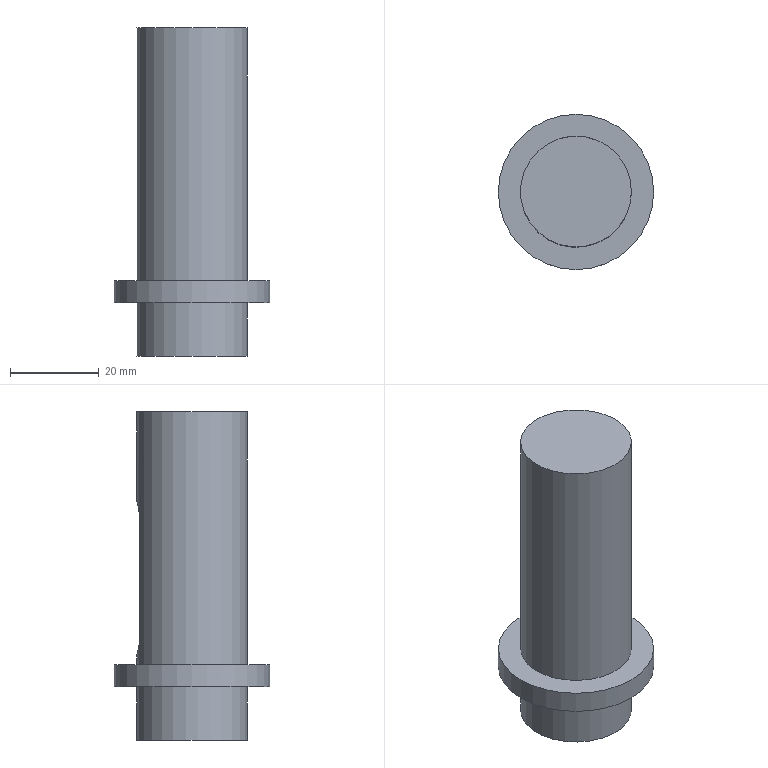Component | NX | MIDDLE_SHAFT | 1 solid | 12 faces | box 35 x 35 x 74 mm | volume 37671 mm3 | plane 7 | cylinder 5 | commonest cylinder face diameters 25 x2 8 x2 35 x1
STEP:
#1=CARTESIAN_POINT('',(0.,0.,0.));
#2=DIRECTION('',(0.,0.,1.));
#3=DIRECTION('',(1.,0.,0.));
#4=AXIS2_PLACEMENT_3D('',#1,#2,#3);
#5=CARTESIAN_POINT('',(-498.675,308.181,-737.));
#6=VERTEX_POINT('',#5);
#7=CARTESIAN_POINT('',(-511.175,308.181,-737.));
#8=DIRECTION('',(0.,0.,1.));
#9=DIRECTION('',(1.,0.,0.));
#10=AXIS2_PLACEMENT_3D('',#7,#8,#9);
#11=CIRCLE('',#10,12.5);
#12=CARTESIAN_POINT('',(-511.175,308.181,-737.));
#13=DIRECTION('',(0.,0.,-1.));
#14=DIRECTION('',(-1.,0.,0.));
#15=AXIS2_PLACEMENT_3D('',#12,#13,#14);
#16=PLANE('',#15);
#17=CARTESIAN_POINT('',(-12.5,0.));
#18=CARTESIAN_POINT('',(-12.5,21.651));
#19=CARTESIAN_POINT('',(6.25,10.825));
#20=CARTESIAN_POINT('',(25.,0.));
#21=CARTESIAN_POINT('',(6.25,-10.825));
#22=CARTESIAN_POINT('',(-12.5,-21.651));
#23=CARTESIAN_POINT('',(-12.5,0.));
#24=(BOUNDED_CURVE()B_SPLINE_CURVE(2,(#17,#18,#19,#20,#21,#22,#23),.UNSPECIFIED.,.T.,.F.)B_SPLINE_CURVE_WITH_KNOTS((1,2,2,2,2,1),(-2.094,0.,2.094,4.189,6.283,8.378),.UNSPECIFIED.)CURVE()GEOMETRIC_REPRESENTATION_ITEM()RATIONAL_B_SPLINE_CURVE((1.,0.5,1.,0.5,1.,0.5,1.))REPRESENTATION_ITEM(''));
#25=(GEOMETRIC_REPRESENTATION_CONTEXT(2)PARAMETRIC_REPRESENTATION_CONTEXT()REPRESENTATION_CONTEXT('',''));
#26=DEFINITIONAL_REPRESENTATION('',(#24),#25);
#27=PCURVE('',#16,#26);
#28=CARTESIAN_POINT('',(-511.175,308.181,-737.));
#29=DIRECTION('',(0.,0.,1.));
#30=DIRECTION('',(1.,0.,0.));
#31=AXIS2_PLACEMENT_3D('',#28,#29,#30);
#32=CYLINDRICAL_SURFACE('',#31,12.5);
#33=CARTESIAN_POINT('',(0.,0.));
#34=DIRECTION('',(1.,0.));
#35=VECTOR('',#34,1.);
#36=LINE('',#33,#35);
#37=(GEOMETRIC_REPRESENTATION_CONTEXT(2)PARAMETRIC_REPRESENTATION_CONTEXT()REPRESENTATION_CONTEXT('',''));
#38=DEFINITIONAL_REPRESENTATION('',(#36),#37);
#39=PCURVE('',#32,#38);
#40=SURFACE_CURVE('',#11,(#27,#39),.PCURVE_S1.);
#41=EDGE_CURVE('',#6,#6,#40,.T.);
#42=ORIENTED_EDGE('',*,*,#41,.F.);
#43=EDGE_LOOP('',(#42));
#44=FACE_BOUND('',#43,.T.);
#45=ADVANCED_FACE('',(#44),#16,.T.);
#46=CARTESIAN_POINT('',(-498.675,308.181,-725.));
#47=VERTEX_POINT('',#46);
#48=CARTESIAN_POINT('',(-511.175,308.181,-725.));
#49=DIRECTION('',(0.,0.,-1.));
#50=DIRECTION('',(1.,0.,0.));
#51=AXIS2_PLACEMENT_3D('',#48,#49,#50);
#52=CIRCLE('',#51,12.5);
#53=CARTESIAN_POINT('',(6.283,12.));
#54=DIRECTION('',(-1.,0.));
#55=VECTOR('',#54,1.);
#56=LINE('',#53,#55);
#57=(GEOMETRIC_REPRESENTATION_CONTEXT(2)PARAMETRIC_REPRESENTATION_CONTEXT()REPRESENTATION_CONTEXT('',''));
#58=DEFINITIONAL_REPRESENTATION('',(#56),#57);
#59=PCURVE('',#32,#58);
#60=CARTESIAN_POINT('',(-511.175,308.181,-725.));
#61=DIRECTION('',(0.,0.,1.));
#62=DIRECTION('',(1.,0.,0.));
#63=AXIS2_PLACEMENT_3D('',#60,#61,#62);
#64=PLANE('',#63);
#65=CARTESIAN_POINT('',(12.5,0.));
#66=CARTESIAN_POINT('',(12.5,-21.651));
#67=CARTESIAN_POINT('',(-6.25,-10.825));
#68=CARTESIAN_POINT('',(-25.,-0.));
#69=CARTESIAN_POINT('',(-6.25,10.825));
#70=CARTESIAN_POINT('',(12.5,21.651));
#71=CARTESIAN_POINT('',(12.5,0.));
#72=(BOUNDED_CURVE()B_SPLINE_CURVE(2,(#65,#66,#67,#68,#69,#70,#71),.UNSPECIFIED.,.T.,.F.)B_SPLINE_CURVE_WITH_KNOTS((1,2,2,2,2,1),(-2.094,0.,2.094,4.189,6.283,8.378),.UNSPECIFIED.)CURVE()GEOMETRIC_REPRESENTATION_ITEM()RATIONAL_B_SPLINE_CURVE((1.,0.5,1.,0.5,1.,0.5,1.))REPRESENTATION_ITEM(''));
#73=(GEOMETRIC_REPRESENTATION_CONTEXT(2)PARAMETRIC_REPRESENTATION_CONTEXT()REPRESENTATION_CONTEXT('',''));
#74=DEFINITIONAL_REPRESENTATION('',(#72),#73);
#75=PCURVE('',#64,#74);
#76=SURFACE_CURVE('',#52,(#59,#75),.PCURVE_S1.);
#77=EDGE_CURVE('',#47,#47,#76,.T.);
#78=ORIENTED_EDGE('',*,*,#77,.T.);
#79=CARTESIAN_POINT('',(-498.675,308.181,-737.));
#80=CARTESIAN_POINT('',(-498.675,308.181,-725.));
#81=B_SPLINE_CURVE_WITH_KNOTS('',1,(#79,#80),.UNSPECIFIED.,.F.,.F.,(2,2),(0.,12.),.PIECEWISE_BEZIER_KNOTS.);
#82=CARTESIAN_POINT('',(0.,0.));
#83=DIRECTION('',(0.,1.));
#84=VECTOR('',#83,1.);
#85=LINE('',#82,#84);
#86=(GEOMETRIC_REPRESENTATION_CONTEXT(2)PARAMETRIC_REPRESENTATION_CONTEXT()REPRESENTATION_CONTEXT('',''));
#87=DEFINITIONAL_REPRESENTATION('',(#85),#86);
#88=PCURVE('',#32,#87);
#89=CARTESIAN_POINT('',(6.283,0.));
#90=DIRECTION('',(0.,1.));
#91=VECTOR('',#90,1.);
#92=LINE('',#89,#91);
#93=(GEOMETRIC_REPRESENTATION_CONTEXT(2)PARAMETRIC_REPRESENTATION_CONTEXT()REPRESENTATION_CONTEXT('',''));
#94=DEFINITIONAL_REPRESENTATION('',(#92),#93);
#95=PCURVE('',#32,#94);
#96=SEAM_CURVE('',#81,(#88,#95),.PCURVE_S1.);
#97=EDGE_CURVE('',#6,#47,#96,.T.);
#98=ORIENTED_EDGE('',*,*,#97,.F.);
#99=ORIENTED_EDGE('',*,*,#41,.T.);
#100=ORIENTED_EDGE('',*,*,#97,.T.);
#101=EDGE_LOOP('',(#78,#98,#99,#100));
#102=FACE_BOUND('',#101,.T.);
#103=ADVANCED_FACE('',(#102),#32,.T.);
#104=CARTESIAN_POINT('',(-493.675,308.181,-720.));
#105=VERTEX_POINT('',#104);
#106=CARTESIAN_POINT('',(-511.175,308.181,-720.));
#107=DIRECTION('',(0.,0.,1.));
#108=DIRECTION('',(1.,0.,0.));
#109=AXIS2_PLACEMENT_3D('',#106,#107,#108);
#110=CIRCLE('',#109,17.5);
#111=CARTESIAN_POINT('',(-511.175,308.181,-720.));
#112=DIRECTION('',(0.,0.,-1.));
#113=DIRECTION('',(-1.,0.,0.));
#114=AXIS2_PLACEMENT_3D('',#111,#112,#113);
#115=CYLINDRICAL_SURFACE('',#114,17.5);
#116=CARTESIAN_POINT('',(9.425,0.));
#117=DIRECTION('',(-1.,0.));
#118=VECTOR('',#117,1.);
#119=LINE('',#116,#118);
#120=(GEOMETRIC_REPRESENTATION_CONTEXT(2)PARAMETRIC_REPRESENTATION_CONTEXT()REPRESENTATION_CONTEXT('',''));
#121=DEFINITIONAL_REPRESENTATION('',(#119),#120);
#122=PCURVE('',#115,#121);
#123=CARTESIAN_POINT('',(-511.175,308.181,-720.));
#124=DIRECTION('',(0.,0.,1.));
#125=DIRECTION('',(1.,0.,0.));
#126=AXIS2_PLACEMENT_3D('',#123,#124,#125);
#127=PLANE('',#126);
#128=CARTESIAN_POINT('',(0.,0.));
#129=DIRECTION('',(1.,0.));
#130=AXIS2_PLACEMENT_2D('',#128,#129);
#131=CIRCLE('',#130,17.5);
#132=(GEOMETRIC_REPRESENTATION_CONTEXT(2)PARAMETRIC_REPRESENTATION_CONTEXT()REPRESENTATION_CONTEXT('',''));
#133=DEFINITIONAL_REPRESENTATION('',(#131),#132);
#134=PCURVE('',#127,#133);
#135=SURFACE_CURVE('',#110,(#122,#134),.PCURVE_S1.);
#136=EDGE_CURVE('',#105,#105,#135,.T.);
#137=ORIENTED_EDGE('',*,*,#136,.F.);
#138=CARTESIAN_POINT('',(-493.675,308.181,-725.));
#139=VERTEX_POINT('',#138);
#140=CARTESIAN_POINT('',(-493.675,308.181,-720.));
#141=CARTESIAN_POINT('',(-493.675,308.181,-725.));
#142=B_SPLINE_CURVE_WITH_KNOTS('',1,(#140,#141),.UNSPECIFIED.,.F.,.F.,(2,2),(0.,5.),.PIECEWISE_BEZIER_KNOTS.);
#143=CARTESIAN_POINT('',(9.425,0.));
#144=DIRECTION('',(0.,1.));
#145=VECTOR('',#144,1.);
#146=LINE('',#143,#145);
#147=(GEOMETRIC_REPRESENTATION_CONTEXT(2)PARAMETRIC_REPRESENTATION_CONTEXT()REPRESENTATION_CONTEXT('',''));
#148=DEFINITIONAL_REPRESENTATION('',(#146),#147);
#149=PCURVE('',#115,#148);
#150=CARTESIAN_POINT('',(3.142,0.));
#151=DIRECTION('',(0.,1.));
#152=VECTOR('',#151,1.);
#153=LINE('',#150,#152);
#154=(GEOMETRIC_REPRESENTATION_CONTEXT(2)PARAMETRIC_REPRESENTATION_CONTEXT()REPRESENTATION_CONTEXT('',''));
#155=DEFINITIONAL_REPRESENTATION('',(#153),#154);
#156=PCURVE('',#115,#155);
#157=SEAM_CURVE('',#142,(#149,#156),.PCURVE_S1.);
#158=EDGE_CURVE('',#105,#139,#157,.T.);
#159=ORIENTED_EDGE('',*,*,#158,.T.);
#160=CARTESIAN_POINT('',(-511.175,308.181,-725.));
#161=DIRECTION('',(0.,0.,1.));
#162=DIRECTION('',(1.,0.,0.));
#163=AXIS2_PLACEMENT_3D('',#160,#161,#162);
#164=CIRCLE('',#163,17.5);
#165=CARTESIAN_POINT('',(9.425,5.));
#166=DIRECTION('',(-1.,0.));
#167=VECTOR('',#166,1.);
#168=LINE('',#165,#167);
#169=(GEOMETRIC_REPRESENTATION_CONTEXT(2)PARAMETRIC_REPRESENTATION_CONTEXT()REPRESENTATION_CONTEXT('',''));
#170=DEFINITIONAL_REPRESENTATION('',(#168),#169);
#171=PCURVE('',#115,#170);
#172=CARTESIAN_POINT('',(0.,0.));
#173=DIRECTION('',(1.,0.));
#174=AXIS2_PLACEMENT_2D('',#172,#173);
#175=CIRCLE('',#174,17.5);
#176=(GEOMETRIC_REPRESENTATION_CONTEXT(2)PARAMETRIC_REPRESENTATION_CONTEXT()REPRESENTATION_CONTEXT('',''));
#177=DEFINITIONAL_REPRESENTATION('',(#175),#176);
#178=PCURVE('',#64,#177);
#179=SURFACE_CURVE('',#164,(#171,#178),.PCURVE_S1.);
#180=EDGE_CURVE('',#139,#139,#179,.T.);
#181=ORIENTED_EDGE('',*,*,#180,.T.);
#182=ORIENTED_EDGE('',*,*,#158,.F.);
#183=EDGE_LOOP('',(#137,#159,#181,#182));
#184=FACE_BOUND('',#183,.T.);
#185=ADVANCED_FACE('',(#184),#115,.T.);
#186=CARTESIAN_POINT('',(-498.675,308.181,-720.));
#187=VERTEX_POINT('',#186);
#188=CARTESIAN_POINT('',(-511.175,308.181,-720.));
#189=DIRECTION('',(0.,0.,1.));
#190=DIRECTION('',(1.,0.,0.));
#191=AXIS2_PLACEMENT_3D('',#188,#189,#190);
#192=CIRCLE('',#191,12.5);
#193=CARTESIAN_POINT('',(0.,0.));
#194=DIRECTION('',(1.,0.));
#195=AXIS2_PLACEMENT_2D('',#193,#194);
#196=CIRCLE('',#195,12.5);
#197=(GEOMETRIC_REPRESENTATION_CONTEXT(2)PARAMETRIC_REPRESENTATION_CONTEXT()REPRESENTATION_CONTEXT('',''));
#198=DEFINITIONAL_REPRESENTATION('',(#196),#197);
#199=PCURVE('',#127,#198);
#200=CARTESIAN_POINT('',(-511.175,308.181,-720.));
#201=DIRECTION('',(0.,0.,1.));
#202=DIRECTION('',(1.,0.,0.));
#203=AXIS2_PLACEMENT_3D('',#200,#201,#202);
#204=CYLINDRICAL_SURFACE('',#203,12.5);
#205=CARTESIAN_POINT('',(0.,0.));
#206=DIRECTION('',(1.,0.));
#207=VECTOR('',#206,1.);
#208=LINE('',#205,#207);
#209=(GEOMETRIC_REPRESENTATION_CONTEXT(2)PARAMETRIC_REPRESENTATION_CONTEXT()REPRESENTATION_CONTEXT('',''));
#210=DEFINITIONAL_REPRESENTATION('',(#208),#209);
#211=PCURVE('',#204,#210);
#212=SURFACE_CURVE('',#192,(#199,#211),.PCURVE_S1.);
#213=EDGE_CURVE('',#187,#187,#212,.T.);
#214=ORIENTED_EDGE('',*,*,#213,.F.);
#215=EDGE_LOOP('',(#214));
#216=FACE_BOUND('',#215,.T.);
#217=ORIENTED_EDGE('',*,*,#136,.T.);
#218=EDGE_LOOP('',(#217));
#219=FACE_BOUND('',#218,.T.);
#220=ADVANCED_FACE('',(#216,#219),#127,.T.);
#221=ORIENTED_EDGE('',*,*,#77,.F.);
#222=EDGE_LOOP('',(#221));
#223=FACE_BOUND('',#222,.T.);
#224=ORIENTED_EDGE('',*,*,#180,.F.);
#225=EDGE_LOOP('',(#224));
#226=FACE_BOUND('',#225,.T.);
#227=ADVANCED_FACE('',(#223,#226),#64,.F.);
#228=CARTESIAN_POINT('',(-498.675,308.181,-663.));
#229=VERTEX_POINT('',#228);
#230=CARTESIAN_POINT('',(-511.175,308.181,-663.));
#231=DIRECTION('',(0.,0.,-1.));
#232=DIRECTION('',(1.,0.,0.));
#233=AXIS2_PLACEMENT_3D('',#230,#231,#232);
#234=CIRCLE('',#233,12.5);
#235=CARTESIAN_POINT('',(-511.175,308.181,-663.));
#236=DIRECTION('',(0.,0.,1.));
#237=DIRECTION('',(1.,0.,0.));
#238=AXIS2_PLACEMENT_3D('',#235,#236,#237);
#239=PLANE('',#238);
#240=CARTESIAN_POINT('',(12.5,0.));
#241=CARTESIAN_POINT('',(12.5,-21.651));
#242=CARTESIAN_POINT('',(-6.25,-10.825));
#243=CARTESIAN_POINT('',(-25.,-0.));
#244=CARTESIAN_POINT('',(-6.25,10.825));
#245=CARTESIAN_POINT('',(12.5,21.651));
#246=CARTESIAN_POINT('',(12.5,0.));
#247=(BOUNDED_CURVE()B_SPLINE_CURVE(2,(#240,#241,#242,#243,#244,#245,#246),.UNSPECIFIED.,.T.,.F.)B_SPLINE_CURVE_WITH_KNOTS((1,2,2,2,2,1),(-2.094,0.,2.094,4.189,6.283,8.378),.UNSPECIFIED.)CURVE()GEOMETRIC_REPRESENTATION_ITEM()RATIONAL_B_SPLINE_CURVE((1.,0.5,1.,0.5,1.,0.5,1.))REPRESENTATION_ITEM(''));
#248=(GEOMETRIC_REPRESENTATION_CONTEXT(2)PARAMETRIC_REPRESENTATION_CONTEXT()REPRESENTATION_CONTEXT('',''));
#249=DEFINITIONAL_REPRESENTATION('',(#247),#248);
#250=PCURVE('',#239,#249);
#251=CARTESIAN_POINT('',(6.283,57.));
#252=DIRECTION('',(-1.,0.));
#253=VECTOR('',#252,1.);
#254=LINE('',#251,#253);
#255=(GEOMETRIC_REPRESENTATION_CONTEXT(2)PARAMETRIC_REPRESENTATION_CONTEXT()REPRESENTATION_CONTEXT('',''));
#256=DEFINITIONAL_REPRESENTATION('',(#254),#255);
#257=PCURVE('',#204,#256);
#258=SURFACE_CURVE('',#234,(#250,#257),.PCURVE_S1.);
#259=EDGE_CURVE('',#229,#229,#258,.T.);
#260=ORIENTED_EDGE('',*,*,#259,.F.);
#261=EDGE_LOOP('',(#260));
#262=FACE_BOUND('',#261,.T.);
#263=ADVANCED_FACE('',(#262),#239,.T.);
#264=ORIENTED_EDGE('',*,*,#259,.T.);
#265=CARTESIAN_POINT('',(-498.675,308.181,-720.));
#266=CARTESIAN_POINT('',(-498.675,308.181,-663.));
#267=B_SPLINE_CURVE_WITH_KNOTS('',1,(#265,#266),.UNSPECIFIED.,.F.,.F.,(2,2),(0.,57.),.PIECEWISE_BEZIER_KNOTS.);
#268=CARTESIAN_POINT('',(0.,0.));
#269=DIRECTION('',(0.,1.));
#270=VECTOR('',#269,1.);
#271=LINE('',#268,#270);
#272=(GEOMETRIC_REPRESENTATION_CONTEXT(2)PARAMETRIC_REPRESENTATION_CONTEXT()REPRESENTATION_CONTEXT('',''));
#273=DEFINITIONAL_REPRESENTATION('',(#271),#272);
#274=PCURVE('',#204,#273);
#275=CARTESIAN_POINT('',(6.283,0.));
#276=DIRECTION('',(0.,1.));
#277=VECTOR('',#276,1.);
#278=LINE('',#275,#277);
#279=(GEOMETRIC_REPRESENTATION_CONTEXT(2)PARAMETRIC_REPRESENTATION_CONTEXT()REPRESENTATION_CONTEXT('',''));
#280=DEFINITIONAL_REPRESENTATION('',(#278),#279);
#281=PCURVE('',#204,#280);
#282=SEAM_CURVE('',#267,(#274,#281),.PCURVE_S1.);
#283=EDGE_CURVE('',#187,#229,#282,.T.);
#284=ORIENTED_EDGE('',*,*,#283,.F.);
#285=ORIENTED_EDGE('',*,*,#213,.T.);
#286=ORIENTED_EDGE('',*,*,#283,.T.);
#287=EDGE_LOOP('',(#264,#284,#285,#286));
#288=FACE_BOUND('',#287,.T.);
#289=CARTESIAN_POINT('',(-507.175,320.024,-687.));
#290=VERTEX_POINT('',#289);
#291=CARTESIAN_POINT('',(-507.175,320.024,-714.));
#292=VERTEX_POINT('',#291);
#293=CARTESIAN_POINT('',(-507.175,320.024,-720.));
#294=DIRECTION('',(0.,0.,-1.));
#295=VECTOR('',#294,1.);
#296=LINE('',#293,#295);
#297=CARTESIAN_POINT('',(1.245,0.));
#298=DIRECTION('',(0.,-1.));
#299=VECTOR('',#298,1.);
#300=LINE('',#297,#299);
#301=(GEOMETRIC_REPRESENTATION_CONTEXT(2)PARAMETRIC_REPRESENTATION_CONTEXT()REPRESENTATION_CONTEXT('',''));
#302=DEFINITIONAL_REPRESENTATION('',(#300),#301);
#303=PCURVE('',#204,#302);
#304=CARTESIAN_POINT('',(-507.175,308.181,-737.));
#305=DIRECTION('',(1.,0.,0.));
#306=DIRECTION('',(0.,0.,-1.));
#307=AXIS2_PLACEMENT_3D('',#304,#305,#306);
#308=PLANE('',#307);
#309=CARTESIAN_POINT('',(-17.,11.843));
#310=DIRECTION('',(1.,0.));
#311=VECTOR('',#310,1.);
#312=LINE('',#309,#311);
#313=(GEOMETRIC_REPRESENTATION_CONTEXT(2)PARAMETRIC_REPRESENTATION_CONTEXT()REPRESENTATION_CONTEXT('',''));
#314=DEFINITIONAL_REPRESENTATION('',(#312),#313);
#315=PCURVE('',#308,#314);
#316=SURFACE_CURVE('',#296,(#303,#315),.PCURVE_S1.);
#317=EDGE_CURVE('',#290,#292,#316,.T.);
#318=ORIENTED_EDGE('',*,*,#317,.F.);
#319=CARTESIAN_POINT('',(-515.175,320.024,-687.));
#320=VERTEX_POINT('',#319);
#321=CARTESIAN_POINT('',(-507.175,320.024,-687.));
#322=CARTESIAN_POINT('',(-507.175,320.024,-686.565));
#323=CARTESIAN_POINT('',(-507.248,320.049,-686.125));
#324=CARTESIAN_POINT('',(-507.387,320.094,-685.715));
#325=CARTESIAN_POINT('',(-507.526,320.138,-685.306));
#326=CARTESIAN_POINT('',(-507.734,320.201,-684.917));
#327=CARTESIAN_POINT('',(-507.994,320.27,-684.576));
#328=CARTESIAN_POINT('',(-508.262,320.34,-684.223));
#329=CARTESIAN_POINT('',(-508.593,320.418,-683.913));
#330=CARTESIAN_POINT('',(-508.963,320.484,-683.668));
#331=CARTESIAN_POINT('',(-509.341,320.552,-683.417));
#332=CARTESIAN_POINT('',(-509.77,320.61,-683.227));
#333=CARTESIAN_POINT('',(-510.215,320.644,-683.117));
#334=CARTESIAN_POINT('',(-510.527,320.668,-683.04));
#335=CARTESIAN_POINT('',(-510.852,320.681,-683.));
#336=CARTESIAN_POINT('',(-511.175,320.681,-683.));
#337=CARTESIAN_POINT('',(-511.611,320.681,-683.));
#338=CARTESIAN_POINT('',(-512.052,320.657,-683.073));
#339=CARTESIAN_POINT('',(-512.462,320.615,-683.213));
#340=CARTESIAN_POINT('',(-512.872,320.573,-683.352));
#341=CARTESIAN_POINT('',(-513.262,320.511,-683.561));
#342=CARTESIAN_POINT('',(-513.604,320.443,-683.821));
#343=CARTESIAN_POINT('',(-513.955,320.374,-684.09));
#344=CARTESIAN_POINT('',(-514.265,320.296,-684.421));
#345=CARTESIAN_POINT('',(-514.509,320.229,-684.79));
#346=CARTESIAN_POINT('',(-514.76,320.159,-685.168));
#347=CARTESIAN_POINT('',(-514.949,320.099,-685.597));
#348=CARTESIAN_POINT('',(-515.059,320.063,-686.041));
#349=CARTESIAN_POINT('',(-515.136,320.038,-686.353));
#350=CARTESIAN_POINT('',(-515.175,320.024,-686.678));
#351=CARTESIAN_POINT('',(-515.175,320.024,-687.));
#352=B_SPLINE_CURVE_WITH_KNOTS('',3,(#321,#322,#323,#324,#325,#326,#327,#328,#329,#330,#331,#332,#333,#334,#335,#336,#337,#338,#339,#340,#341,#342,#343,#344,#345,#346,#347,#348,#349,#350,#351),.UNSPECIFIED.,.F.,.F.,(4,3,3,3,3,3,3,3,3,3,4),(0.,0.1037,0.2071,0.314,0.4235,0.5,0.6038,0.7074,0.8141,0.9237,1.),.UNSPECIFIED.);
#353=CARTESIAN_POINT('',(1.245,33.));
#354=CARTESIAN_POINT('',(1.245,33.095));
#355=CARTESIAN_POINT('',(1.246,33.286));
#356=CARTESIAN_POINT('',(1.248,33.573));
#357=CARTESIAN_POINT('',(1.253,33.856));
#358=CARTESIAN_POINT('',(1.259,34.134));
#359=CARTESIAN_POINT('',(1.266,34.404));
#360=CARTESIAN_POINT('',(1.275,34.667));
#361=CARTESIAN_POINT('',(1.286,34.923));
#362=CARTESIAN_POINT('',(1.298,35.168));
#363=CARTESIAN_POINT('',(1.312,35.401));
#364=CARTESIAN_POINT('',(1.326,35.621));
#365=CARTESIAN_POINT('',(1.342,35.829));
#366=CARTESIAN_POINT('',(1.359,36.023));
#367=CARTESIAN_POINT('',(1.377,36.202));
#368=CARTESIAN_POINT('',(1.396,36.364));
#369=CARTESIAN_POINT('',(1.416,36.509));
#370=CARTESIAN_POINT('',(1.437,36.637));
#371=CARTESIAN_POINT('',(1.458,36.747));
#372=CARTESIAN_POINT('',(1.48,36.839));
#373=CARTESIAN_POINT('',(1.502,36.91));
#374=CARTESIAN_POINT('',(1.525,36.962));
#375=CARTESIAN_POINT('',(1.548,36.993));
#376=CARTESIAN_POINT('',(1.571,37.004));
#377=CARTESIAN_POINT('',(1.594,36.993));
#378=CARTESIAN_POINT('',(1.617,36.962));
#379=CARTESIAN_POINT('',(1.639,36.91));
#380=CARTESIAN_POINT('',(1.662,36.839));
#381=CARTESIAN_POINT('',(1.683,36.749));
#382=CARTESIAN_POINT('',(1.705,36.639));
#383=CARTESIAN_POINT('',(1.725,36.511));
#384=CARTESIAN_POINT('',(1.745,36.365));
#385=CARTESIAN_POINT('',(1.764,36.203));
#386=CARTESIAN_POINT('',(1.782,36.025));
#387=CARTESIAN_POINT('',(1.799,35.831));
#388=CARTESIAN_POINT('',(1.815,35.623));
#389=CARTESIAN_POINT('',(1.83,35.402));
#390=CARTESIAN_POINT('',(1.843,35.17));
#391=CARTESIAN_POINT('',(1.855,34.926));
#392=CARTESIAN_POINT('',(1.866,34.671));
#393=CARTESIAN_POINT('',(1.875,34.407));
#394=CARTESIAN_POINT('',(1.883,34.136));
#395=CARTESIAN_POINT('',(1.889,33.86));
#396=CARTESIAN_POINT('',(1.893,33.576));
#397=CARTESIAN_POINT('',(1.896,33.288));
#398=CARTESIAN_POINT('',(1.897,33.096));
#399=CARTESIAN_POINT('',(1.897,33.));
#400=B_SPLINE_CURVE_WITH_KNOTS('',3,(#353,#354,#355,#356,#357,#358,#359,#360,#361,#362,#363,#364,#365,#366,#367,#368,#369,#370,#371,#372,#373,#374,#375,#376,#377,#378,#379,#380,#381,#382,#383,#384,#385,#386,#387,#388,#389,#390,#391,#392,#393,#394,#395,#396,#397,#398,#399),.UNSPECIFIED.,.F.,.F.,(4,1,1,1,1,1,1,1,1,1,1,1,1,1,1,1,1,1,1,1,1,1,1,1,1,1,1,1,1,1,1,1,1,1,1,1,1,1,1,1,1,1,1,1,4),(0.,0.02273,0.04545,0.06818,0.09091,0.1136,0.1364,0.1591,0.1818,0.2045,0.2273,0.25,0.2727,0.2955,0.3182,0.3409,0.3636,0.3864,0.4091,0.4318,0.4545,0.4773,0.5,0.5227,0.5455,0.5682,0.5909,0.6136,0.6364,0.6591,0.6818,0.7045,0.7273,0.75,0.7727,0.7955,0.8182,0.8409,0.8636,0.8864,0.9091,0.9318,0.9545,0.9773,1.),.QUASI_UNIFORM_KNOTS.);
#401=(GEOMETRIC_REPRESENTATION_CONTEXT(2)PARAMETRIC_REPRESENTATION_CONTEXT()REPRESENTATION_CONTEXT('',''));
#402=DEFINITIONAL_REPRESENTATION('',(#400),#401);
#403=PCURVE('',#204,#402);
#404=CARTESIAN_POINT('',(-511.175,308.181,-687.));
#405=DIRECTION('',(0.,1.,0.));
#406=DIRECTION('',(0.,0.,1.));
#407=AXIS2_PLACEMENT_3D('',#404,#405,#406);
#408=CYLINDRICAL_SURFACE('',#407,4.);
#409=CARTESIAN_POINT('',(1.571,11.843));
#410=CARTESIAN_POINT('',(1.547,11.843));
#411=CARTESIAN_POINT('',(1.499,11.845));
#412=CARTESIAN_POINT('',(1.427,11.856));
#413=CARTESIAN_POINT('',(1.355,11.873));
#414=CARTESIAN_POINT('',(1.284,11.896));
#415=CARTESIAN_POINT('',(1.213,11.925));
#416=CARTESIAN_POINT('',(1.141,11.959));
#417=CARTESIAN_POINT('',(1.07,11.997));
#418=CARTESIAN_POINT('',(0.9985,12.039));
#419=CARTESIAN_POINT('',(0.9276,12.083));
#420=CARTESIAN_POINT('',(0.857,12.129));
#421=CARTESIAN_POINT('',(0.7859,12.175));
#422=CARTESIAN_POINT('',(0.7149,12.222));
#423=CARTESIAN_POINT('',(0.6438,12.268));
#424=CARTESIAN_POINT('',(0.5731,12.311));
#425=CARTESIAN_POINT('',(0.5022,12.351));
#426=CARTESIAN_POINT('',(0.4308,12.388));
#427=CARTESIAN_POINT('',(0.3593,12.421));
#428=CARTESIAN_POINT('',(0.2878,12.449));
#429=CARTESIAN_POINT('',(0.2165,12.471));
#430=CARTESIAN_POINT('',(0.1443,12.488));
#431=CARTESIAN_POINT('',(0.07209,12.498));
#432=CARTESIAN_POINT('',(-0.0001412,12.501));
#433=CARTESIAN_POINT('',(-0.07158,12.498));
#434=CARTESIAN_POINT('',(-0.1436,12.488));
#435=CARTESIAN_POINT('',(-0.2155,12.472));
#436=CARTESIAN_POINT('',(-0.2872,12.449));
#437=CARTESIAN_POINT('',(-0.3583,12.422));
#438=CARTESIAN_POINT('',(-0.4297,12.389));
#439=CARTESIAN_POINT('',(-0.5012,12.352));
#440=CARTESIAN_POINT('',(-0.5725,12.311));
#441=CARTESIAN_POINT('',(-0.6434,12.268));
#442=CARTESIAN_POINT('',(-0.7141,12.223));
#443=CARTESIAN_POINT('',(-0.7851,12.176));
#444=CARTESIAN_POINT('',(-0.8562,12.129));
#445=CARTESIAN_POINT('',(-0.9272,12.083));
#446=CARTESIAN_POINT('',(-0.9979,12.039));
#447=CARTESIAN_POINT('',(-1.069,11.998));
#448=CARTESIAN_POINT('',(-1.14,11.959));
#449=CARTESIAN_POINT('',(-1.212,11.925));
#450=CARTESIAN_POINT('',(-1.283,11.896));
#451=CARTESIAN_POINT('',(-1.354,11.873));
#452=CARTESIAN_POINT('',(-1.427,11.856));
#453=CARTESIAN_POINT('',(-1.499,11.845));
#454=CARTESIAN_POINT('',(-1.547,11.843));
#455=CARTESIAN_POINT('',(-1.571,11.843));
#456=B_SPLINE_CURVE_WITH_KNOTS('',3,(#409,#410,#411,#412,#413,#414,#415,#416,#417,#418,#419,#420,#421,#422,#423,#424,#425,#426,#427,#428,#429,#430,#431,#432,#433,#434,#435,#436,#437,#438,#439,#440,#441,#442,#443,#444,#445,#446,#447,#448,#449,#450,#451,#452,#453,#454,#455),.UNSPECIFIED.,.F.,.F.,(4,1,1,1,1,1,1,1,1,1,1,1,1,1,1,1,1,1,1,1,1,1,1,1,1,1,1,1,1,1,1,1,1,1,1,1,1,1,1,1,1,1,1,1,4),(0.,0.02273,0.04545,0.06818,0.09091,0.1136,0.1364,0.1591,0.1818,0.2045,0.2273,0.25,0.2727,0.2955,0.3182,0.3409,0.3636,0.3864,0.4091,0.4318,0.4545,0.4773,0.5,0.5227,0.5455,0.5682,0.5909,0.6136,0.6364,0.6591,0.6818,0.7045,0.7273,0.75,0.7727,0.7955,0.8182,0.8409,0.8636,0.8864,0.9091,0.9318,0.9545,0.9773,1.),.QUASI_UNIFORM_KNOTS.);
#457=(GEOMETRIC_REPRESENTATION_CONTEXT(2)PARAMETRIC_REPRESENTATION_CONTEXT()REPRESENTATION_CONTEXT('',''));
#458=DEFINITIONAL_REPRESENTATION('',(#456),#457);
#459=PCURVE('',#408,#458);
#460=SURFACE_CURVE('',#352,(#403,#459),.PCURVE_S1.);
#461=EDGE_CURVE('',#290,#320,#460,.T.);
#462=ORIENTED_EDGE('',*,*,#461,.T.);
#463=CARTESIAN_POINT('',(-515.175,320.024,-714.));
#464=VERTEX_POINT('',#463);
#465=CARTESIAN_POINT('',(-515.175,320.024,-720.));
#466=DIRECTION('',(0.,0.,-1.));
#467=VECTOR('',#466,1.);
#468=LINE('',#465,#467);
#469=CARTESIAN_POINT('',(1.897,0.));
#470=DIRECTION('',(0.,-1.));
#471=VECTOR('',#470,1.);
#472=LINE('',#469,#471);
#473=(GEOMETRIC_REPRESENTATION_CONTEXT(2)PARAMETRIC_REPRESENTATION_CONTEXT()REPRESENTATION_CONTEXT('',''));
#474=DEFINITIONAL_REPRESENTATION('',(#472),#473);
#475=PCURVE('',#204,#474);
#476=CARTESIAN_POINT('',(-515.175,308.181,-737.));
#477=DIRECTION('',(1.,0.,0.));
#478=DIRECTION('',(0.,0.,-1.));
#479=AXIS2_PLACEMENT_3D('',#476,#477,#478);
#480=PLANE('',#479);
#481=CARTESIAN_POINT('',(-17.,11.843));
#482=DIRECTION('',(1.,0.));
#483=VECTOR('',#482,1.);
#484=LINE('',#481,#483);
#485=(GEOMETRIC_REPRESENTATION_CONTEXT(2)PARAMETRIC_REPRESENTATION_CONTEXT()REPRESENTATION_CONTEXT('',''));
#486=DEFINITIONAL_REPRESENTATION('',(#484),#485);
#487=PCURVE('',#480,#486);
#488=SURFACE_CURVE('',#468,(#475,#487),.PCURVE_S1.);
#489=EDGE_CURVE('',#320,#464,#488,.T.);
#490=ORIENTED_EDGE('',*,*,#489,.T.);
#491=CARTESIAN_POINT('',(-515.175,320.024,-714.));
#492=CARTESIAN_POINT('',(-515.175,320.024,-714.435));
#493=CARTESIAN_POINT('',(-515.102,320.049,-714.875));
#494=CARTESIAN_POINT('',(-514.963,320.094,-715.285));
#495=CARTESIAN_POINT('',(-514.824,320.138,-715.694));
#496=CARTESIAN_POINT('',(-514.617,320.201,-716.083));
#497=CARTESIAN_POINT('',(-514.357,320.27,-716.424));
#498=CARTESIAN_POINT('',(-514.088,320.34,-716.777));
#499=CARTESIAN_POINT('',(-513.757,320.418,-717.087));
#500=CARTESIAN_POINT('',(-513.388,320.484,-717.332));
#501=CARTESIAN_POINT('',(-513.01,320.552,-717.583));
#502=CARTESIAN_POINT('',(-512.58,320.61,-717.773));
#503=CARTESIAN_POINT('',(-512.136,320.644,-717.883));
#504=CARTESIAN_POINT('',(-511.823,320.668,-717.96));
#505=CARTESIAN_POINT('',(-511.498,320.681,-718.));
#506=CARTESIAN_POINT('',(-511.175,320.681,-718.));
#507=CARTESIAN_POINT('',(-510.74,320.681,-718.));
#508=CARTESIAN_POINT('',(-510.299,320.657,-717.927));
#509=CARTESIAN_POINT('',(-509.888,320.615,-717.787));
#510=CARTESIAN_POINT('',(-509.478,320.573,-717.648));
#511=CARTESIAN_POINT('',(-509.088,320.511,-717.439));
#512=CARTESIAN_POINT('',(-508.747,320.443,-717.179));
#513=CARTESIAN_POINT('',(-508.396,320.374,-716.91));
#514=CARTESIAN_POINT('',(-508.086,320.296,-716.579));
#515=CARTESIAN_POINT('',(-507.842,320.229,-716.21));
#516=CARTESIAN_POINT('',(-507.591,320.159,-715.832));
#517=CARTESIAN_POINT('',(-507.402,320.099,-715.403));
#518=CARTESIAN_POINT('',(-507.292,320.063,-714.959));
#519=CARTESIAN_POINT('',(-507.215,320.038,-714.647));
#520=CARTESIAN_POINT('',(-507.175,320.024,-714.322));
#521=CARTESIAN_POINT('',(-507.175,320.024,-714.));
#522=B_SPLINE_CURVE_WITH_KNOTS('',3,(#491,#492,#493,#494,#495,#496,#497,#498,#499,#500,#501,#502,#503,#504,#505,#506,#507,#508,#509,#510,#511,#512,#513,#514,#515,#516,#517,#518,#519,#520,#521),.UNSPECIFIED.,.F.,.F.,(4,3,3,3,3,3,3,3,3,3,4),(0.,0.1037,0.2071,0.314,0.4235,0.5,0.6038,0.7074,0.8141,0.9237,1.),.UNSPECIFIED.);
#523=CARTESIAN_POINT('',(1.897,6.));
#524=CARTESIAN_POINT('',(1.897,5.905));
#525=CARTESIAN_POINT('',(1.896,5.714));
#526=CARTESIAN_POINT('',(1.893,5.427));
#527=CARTESIAN_POINT('',(1.889,5.144));
#528=CARTESIAN_POINT('',(1.883,4.866));
#529=CARTESIAN_POINT('',(1.875,4.596));
#530=CARTESIAN_POINT('',(1.866,4.333));
#531=CARTESIAN_POINT('',(1.856,4.077));
#532=CARTESIAN_POINT('',(1.843,3.832));
#533=CARTESIAN_POINT('',(1.83,3.599));
#534=CARTESIAN_POINT('',(1.815,3.379));
#535=CARTESIAN_POINT('',(1.799,3.171));
#536=CARTESIAN_POINT('',(1.782,2.977));
#537=CARTESIAN_POINT('',(1.764,2.798));
#538=CARTESIAN_POINT('',(1.745,2.636));
#539=CARTESIAN_POINT('',(1.726,2.491));
#540=CARTESIAN_POINT('',(1.705,2.363));
#541=CARTESIAN_POINT('',(1.684,2.253));
#542=CARTESIAN_POINT('',(1.662,2.161));
#543=CARTESIAN_POINT('',(1.64,2.09));
#544=CARTESIAN_POINT('',(1.617,2.038));
#545=CARTESIAN_POINT('',(1.594,2.007));
#546=CARTESIAN_POINT('',(1.571,1.996));
#547=CARTESIAN_POINT('',(1.548,2.007));
#548=CARTESIAN_POINT('',(1.525,2.038));
#549=CARTESIAN_POINT('',(1.502,2.09));
#550=CARTESIAN_POINT('',(1.48,2.161));
#551=CARTESIAN_POINT('',(1.458,2.251));
#552=CARTESIAN_POINT('',(1.437,2.361));
#553=CARTESIAN_POINT('',(1.416,2.489));
#554=CARTESIAN_POINT('',(1.396,2.635));
#555=CARTESIAN_POINT('',(1.377,2.797));
#556=CARTESIAN_POINT('',(1.359,2.975));
#557=CARTESIAN_POINT('',(1.342,3.169));
#558=CARTESIAN_POINT('',(1.326,3.377));
#559=CARTESIAN_POINT('',(1.312,3.598));
#560=CARTESIAN_POINT('',(1.298,3.83));
#561=CARTESIAN_POINT('',(1.286,4.074));
#562=CARTESIAN_POINT('',(1.276,4.329));
#563=CARTESIAN_POINT('',(1.266,4.593));
#564=CARTESIAN_POINT('',(1.259,4.864));
#565=CARTESIAN_POINT('',(1.253,5.14));
#566=CARTESIAN_POINT('',(1.248,5.424));
#567=CARTESIAN_POINT('',(1.246,5.712));
#568=CARTESIAN_POINT('',(1.245,5.904));
#569=CARTESIAN_POINT('',(1.245,6.));
#570=B_SPLINE_CURVE_WITH_KNOTS('',3,(#523,#524,#525,#526,#527,#528,#529,#530,#531,#532,#533,#534,#535,#536,#537,#538,#539,#540,#541,#542,#543,#544,#545,#546,#547,#548,#549,#550,#551,#552,#553,#554,#555,#556,#557,#558,#559,#560,#561,#562,#563,#564,#565,#566,#567,#568,#569),.UNSPECIFIED.,.F.,.F.,(4,1,1,1,1,1,1,1,1,1,1,1,1,1,1,1,1,1,1,1,1,1,1,1,1,1,1,1,1,1,1,1,1,1,1,1,1,1,1,1,1,1,1,1,4),(0.,0.02273,0.04545,0.06818,0.09091,0.1136,0.1364,0.1591,0.1818,0.2045,0.2273,0.25,0.2727,0.2955,0.3182,0.3409,0.3636,0.3864,0.4091,0.4318,0.4545,0.4773,0.5,0.5227,0.5455,0.5682,0.5909,0.6136,0.6364,0.6591,0.6818,0.7045,0.7273,0.75,0.7727,0.7955,0.8182,0.8409,0.8636,0.8864,0.9091,0.9318,0.9545,0.9773,1.),.QUASI_UNIFORM_KNOTS.);
#571=(GEOMETRIC_REPRESENTATION_CONTEXT(2)PARAMETRIC_REPRESENTATION_CONTEXT()REPRESENTATION_CONTEXT('',''));
#572=DEFINITIONAL_REPRESENTATION('',(#570),#571);
#573=PCURVE('',#204,#572);
#574=CARTESIAN_POINT('',(-511.175,316.681,-714.));
#575=DIRECTION('',(0.,1.,0.));
#576=DIRECTION('',(0.,-0.,1.));
#577=AXIS2_PLACEMENT_3D('',#574,#575,#576);
#578=CYLINDRICAL_SURFACE('',#577,4.);
#579=CARTESIAN_POINT('',(4.712,3.343));
#580=CARTESIAN_POINT('',(4.689,3.343));
#581=CARTESIAN_POINT('',(4.641,3.345));
#582=CARTESIAN_POINT('',(4.569,3.356));
#583=CARTESIAN_POINT('',(4.497,3.373));
#584=CARTESIAN_POINT('',(4.425,3.396));
#585=CARTESIAN_POINT('',(4.354,3.425));
#586=CARTESIAN_POINT('',(4.283,3.459));
#587=CARTESIAN_POINT('',(4.211,3.497));
#588=CARTESIAN_POINT('',(4.14,3.539));
#589=CARTESIAN_POINT('',(4.069,3.583));
#590=CARTESIAN_POINT('',(3.999,3.629));
#591=CARTESIAN_POINT('',(3.928,3.675));
#592=CARTESIAN_POINT('',(3.856,3.722));
#593=CARTESIAN_POINT('',(3.785,3.768));
#594=CARTESIAN_POINT('',(3.715,3.811));
#595=CARTESIAN_POINT('',(3.644,3.851));
#596=CARTESIAN_POINT('',(3.572,3.888));
#597=CARTESIAN_POINT('',(3.501,3.921));
#598=CARTESIAN_POINT('',(3.429,3.949));
#599=CARTESIAN_POINT('',(3.358,3.971));
#600=CARTESIAN_POINT('',(3.286,3.988));
#601=CARTESIAN_POINT('',(3.214,3.998));
#602=CARTESIAN_POINT('',(3.141,4.001));
#603=CARTESIAN_POINT('',(3.07,3.998));
#604=CARTESIAN_POINT('',(2.998,3.988));
#605=CARTESIAN_POINT('',(2.926,3.972));
#606=CARTESIAN_POINT('',(2.854,3.949));
#607=CARTESIAN_POINT('',(2.783,3.922));
#608=CARTESIAN_POINT('',(2.712,3.889));
#609=CARTESIAN_POINT('',(2.64,3.852));
#610=CARTESIAN_POINT('',(2.569,3.811));
#611=CARTESIAN_POINT('',(2.498,3.768));
#612=CARTESIAN_POINT('',(2.428,3.723));
#613=CARTESIAN_POINT('',(2.357,3.676));
#614=CARTESIAN_POINT('',(2.285,3.629));
#615=CARTESIAN_POINT('',(2.214,3.583));
#616=CARTESIAN_POINT('',(2.144,3.539));
#617=CARTESIAN_POINT('',(2.073,3.498));
#618=CARTESIAN_POINT('',(2.001,3.459));
#619=CARTESIAN_POINT('',(1.93,3.425));
#620=CARTESIAN_POINT('',(1.859,3.396));
#621=CARTESIAN_POINT('',(1.787,3.373));
#622=CARTESIAN_POINT('',(1.715,3.356));
#623=CARTESIAN_POINT('',(1.643,3.345));
#624=CARTESIAN_POINT('',(1.595,3.343));
#625=CARTESIAN_POINT('',(1.571,3.343));
#626=B_SPLINE_CURVE_WITH_KNOTS('',3,(#579,#580,#581,#582,#583,#584,#585,#586,#587,#588,#589,#590,#591,#592,#593,#594,#595,#596,#597,#598,#599,#600,#601,#602,#603,#604,#605,#606,#607,#608,#609,#610,#611,#612,#613,#614,#615,#616,#617,#618,#619,#620,#621,#622,#623,#624,#625),.UNSPECIFIED.,.F.,.F.,(4,1,1,1,1,1,1,1,1,1,1,1,1,1,1,1,1,1,1,1,1,1,1,1,1,1,1,1,1,1,1,1,1,1,1,1,1,1,1,1,1,1,1,1,4),(0.,0.02273,0.04545,0.06818,0.09091,0.1136,0.1364,0.1591,0.1818,0.2045,0.2273,0.25,0.2727,0.2955,0.3182,0.3409,0.3636,0.3864,0.4091,0.4318,0.4545,0.4773,0.5,0.5227,0.5455,0.5682,0.5909,0.6136,0.6364,0.6591,0.6818,0.7045,0.7273,0.75,0.7727,0.7955,0.8182,0.8409,0.8636,0.8864,0.9091,0.9318,0.9545,0.9773,1.),.QUASI_UNIFORM_KNOTS.);
#627=(GEOMETRIC_REPRESENTATION_CONTEXT(2)PARAMETRIC_REPRESENTATION_CONTEXT()REPRESENTATION_CONTEXT('',''));
#628=DEFINITIONAL_REPRESENTATION('',(#626),#627);
#629=PCURVE('',#578,#628);
#630=SURFACE_CURVE('',#522,(#573,#629),.PCURVE_S1.);
#631=EDGE_CURVE('',#464,#292,#630,.T.);
#632=ORIENTED_EDGE('',*,*,#631,.T.);
#633=EDGE_LOOP('',(#318,#462,#490,#632));
#634=FACE_BOUND('',#633,.T.);
#635=ADVANCED_FACE('',(#288,#634),#204,.T.);
#636=CARTESIAN_POINT('',(-507.175,316.681,-714.));
#637=VERTEX_POINT('',#636);
#638=CARTESIAN_POINT('',(-507.175,316.681,-687.));
#639=VERTEX_POINT('',#638);
#640=CARTESIAN_POINT('',(-507.175,316.681,-683.));
#641=DIRECTION('',(0.,-0.,1.));
#642=VECTOR('',#641,1.);
#643=LINE('',#640,#642);
#644=CARTESIAN_POINT('',(-507.175,316.681,-683.));
#645=DIRECTION('',(0.,1.,0.));
#646=DIRECTION('',(0.,-0.,1.));
#647=AXIS2_PLACEMENT_3D('',#644,#645,#646);
#648=PLANE('',#647);
#649=CARTESIAN_POINT('',(0.,0.));
#650=DIRECTION('',(1.,0.));
#651=VECTOR('',#650,1.);
#652=LINE('',#649,#651);
#653=(GEOMETRIC_REPRESENTATION_CONTEXT(2)PARAMETRIC_REPRESENTATION_CONTEXT()REPRESENTATION_CONTEXT('',''));
#654=DEFINITIONAL_REPRESENTATION('',(#652),#653);
#655=PCURVE('',#648,#654);
#656=CARTESIAN_POINT('',(-54.,8.5));
#657=DIRECTION('',(-1.,-0.));
#658=VECTOR('',#657,1.);
#659=LINE('',#656,#658);
#660=(GEOMETRIC_REPRESENTATION_CONTEXT(2)PARAMETRIC_REPRESENTATION_CONTEXT()REPRESENTATION_CONTEXT('',''));
#661=DEFINITIONAL_REPRESENTATION('',(#659),#660);
#662=PCURVE('',#308,#661);
#663=SURFACE_CURVE('',#643,(#655,#662),.PCURVE_S1.);
#664=EDGE_CURVE('',#637,#639,#663,.T.);
#665=ORIENTED_EDGE('',*,*,#664,.F.);
#666=CARTESIAN_POINT('',(-515.175,316.681,-714.));
#667=VERTEX_POINT('',#666);
#668=CARTESIAN_POINT('',(-511.175,316.681,-714.));
#669=DIRECTION('',(0.,1.,0.));
#670=DIRECTION('',(0.,-0.,1.));
#671=AXIS2_PLACEMENT_3D('',#668,#669,#670);
#672=CIRCLE('',#671,4.);
#673=CARTESIAN_POINT('',(-31.,-4.));
#674=DIRECTION('',(1.,0.));
#675=AXIS2_PLACEMENT_2D('',#673,#674);
#676=CIRCLE('',#675,4.);
#677=(GEOMETRIC_REPRESENTATION_CONTEXT(2)PARAMETRIC_REPRESENTATION_CONTEXT()REPRESENTATION_CONTEXT('',''));
#678=DEFINITIONAL_REPRESENTATION('',(#676),#677);
#679=PCURVE('',#648,#678);
#680=CARTESIAN_POINT('',(0.,0.));
#681=DIRECTION('',(1.,0.));
#682=VECTOR('',#681,1.);
#683=LINE('',#680,#682);
#684=(GEOMETRIC_REPRESENTATION_CONTEXT(2)PARAMETRIC_REPRESENTATION_CONTEXT()REPRESENTATION_CONTEXT('',''));
#685=DEFINITIONAL_REPRESENTATION('',(#683),#684);
#686=PCURVE('',#578,#685);
#687=SURFACE_CURVE('',#672,(#679,#686),.PCURVE_S1.);
#688=EDGE_CURVE('',#637,#667,#687,.T.);
#689=ORIENTED_EDGE('',*,*,#688,.T.);
#690=CARTESIAN_POINT('',(-515.175,316.681,-687.));
#691=VERTEX_POINT('',#690);
#692=CARTESIAN_POINT('',(-515.175,316.681,-683.));
#693=DIRECTION('',(0.,-0.,1.));
#694=VECTOR('',#693,1.);
#695=LINE('',#692,#694);
#696=CARTESIAN_POINT('',(0.,-8.));
#697=DIRECTION('',(1.,0.));
#698=VECTOR('',#697,1.);
#699=LINE('',#696,#698);
#700=(GEOMETRIC_REPRESENTATION_CONTEXT(2)PARAMETRIC_REPRESENTATION_CONTEXT()REPRESENTATION_CONTEXT('',''));
#701=DEFINITIONAL_REPRESENTATION('',(#699),#700);
#702=PCURVE('',#648,#701);
#703=CARTESIAN_POINT('',(-54.,8.5));
#704=DIRECTION('',(-1.,-0.));
#705=VECTOR('',#704,1.);
#706=LINE('',#703,#705);
#707=(GEOMETRIC_REPRESENTATION_CONTEXT(2)PARAMETRIC_REPRESENTATION_CONTEXT()REPRESENTATION_CONTEXT('',''));
#708=DEFINITIONAL_REPRESENTATION('',(#706),#707);
#709=PCURVE('',#480,#708);
#710=SURFACE_CURVE('',#695,(#702,#709),.PCURVE_S1.);
#711=EDGE_CURVE('',#667,#691,#710,.T.);
#712=ORIENTED_EDGE('',*,*,#711,.T.);
#713=CARTESIAN_POINT('',(-511.175,316.681,-687.));
#714=DIRECTION('',(0.,1.,0.));
#715=DIRECTION('',(0.,-0.,1.));
#716=AXIS2_PLACEMENT_3D('',#713,#714,#715);
#717=CIRCLE('',#716,4.);
#718=CARTESIAN_POINT('',(-4.,-4.));
#719=DIRECTION('',(1.,0.));
#720=AXIS2_PLACEMENT_2D('',#718,#719);
#721=CIRCLE('',#720,4.);
#722=(GEOMETRIC_REPRESENTATION_CONTEXT(2)PARAMETRIC_REPRESENTATION_CONTEXT()REPRESENTATION_CONTEXT('',''));
#723=DEFINITIONAL_REPRESENTATION('',(#721),#722);
#724=PCURVE('',#648,#723);
#725=CARTESIAN_POINT('',(-6.283,8.5));
#726=DIRECTION('',(1.,0.));
#727=VECTOR('',#726,1.);
#728=LINE('',#725,#727);
#729=(GEOMETRIC_REPRESENTATION_CONTEXT(2)PARAMETRIC_REPRESENTATION_CONTEXT()REPRESENTATION_CONTEXT('',''));
#730=DEFINITIONAL_REPRESENTATION('',(#728),#729);
#731=PCURVE('',#408,#730);
#732=SURFACE_CURVE('',#717,(#724,#731),.PCURVE_S1.);
#733=EDGE_CURVE('',#691,#639,#732,.T.);
#734=ORIENTED_EDGE('',*,*,#733,.T.);
#735=EDGE_LOOP('',(#665,#689,#712,#734));
#736=FACE_BOUND('',#735,.T.);
#737=ADVANCED_FACE('',(#736),#648,.T.);
#738=ORIENTED_EDGE('',*,*,#317,.T.);
#739=CARTESIAN_POINT('',(-507.175,308.181,-714.));
#740=DIRECTION('',(0.,-1.,-0.));
#741=VECTOR('',#740,1.);
#742=LINE('',#739,#741);
#743=CARTESIAN_POINT('',(-23.,0.));
#744=DIRECTION('',(0.,-1.));
#745=VECTOR('',#744,1.);
#746=LINE('',#743,#745);
#747=(GEOMETRIC_REPRESENTATION_CONTEXT(2)PARAMETRIC_REPRESENTATION_CONTEXT()REPRESENTATION_CONTEXT('',''));
#748=DEFINITIONAL_REPRESENTATION('',(#746),#747);
#749=PCURVE('',#308,#748);
#750=CARTESIAN_POINT('',(1.571,-8.5));
#751=DIRECTION('',(-0.,-1.));
#752=VECTOR('',#751,1.);
#753=LINE('',#750,#752);
#754=(GEOMETRIC_REPRESENTATION_CONTEXT(2)PARAMETRIC_REPRESENTATION_CONTEXT()REPRESENTATION_CONTEXT('',''));
#755=DEFINITIONAL_REPRESENTATION('',(#753),#754);
#756=PCURVE('',#578,#755);
#757=SURFACE_CURVE('',#742,(#749,#756),.PCURVE_S1.);
#758=EDGE_CURVE('',#292,#637,#757,.T.);
#759=ORIENTED_EDGE('',*,*,#758,.T.);
#760=ORIENTED_EDGE('',*,*,#664,.T.);
#761=CARTESIAN_POINT('',(-507.175,308.181,-687.));
#762=DIRECTION('',(0.,1.,0.));
#763=VECTOR('',#762,1.);
#764=LINE('',#761,#763);
#765=CARTESIAN_POINT('',(-50.,0.));
#766=DIRECTION('',(0.,1.));
#767=VECTOR('',#766,1.);
#768=LINE('',#765,#767);
#769=(GEOMETRIC_REPRESENTATION_CONTEXT(2)PARAMETRIC_REPRESENTATION_CONTEXT()REPRESENTATION_CONTEXT('',''));
#770=DEFINITIONAL_REPRESENTATION('',(#768),#769);
#771=PCURVE('',#308,#770);
#772=CARTESIAN_POINT('',(1.571,0.));
#773=DIRECTION('',(0.,1.));
#774=VECTOR('',#773,1.);
#775=LINE('',#772,#774);
#776=(GEOMETRIC_REPRESENTATION_CONTEXT(2)PARAMETRIC_REPRESENTATION_CONTEXT()REPRESENTATION_CONTEXT('',''));
#777=DEFINITIONAL_REPRESENTATION('',(#775),#776);
#778=PCURVE('',#408,#777);
#779=SURFACE_CURVE('',#764,(#771,#778),.PCURVE_S1.);
#780=EDGE_CURVE('',#639,#290,#779,.T.);
#781=ORIENTED_EDGE('',*,*,#780,.T.);
#782=EDGE_LOOP('',(#738,#759,#760,#781));
#783=FACE_BOUND('',#782,.T.);
#784=ADVANCED_FACE('',(#783),#308,.F.);
#785=ORIENTED_EDGE('',*,*,#711,.F.);
#786=CARTESIAN_POINT('',(-515.175,320.024,-714.));
#787=DIRECTION('',(0.,1.,0.));
#788=VECTOR('',#787,1.);
#789=LINE('',#786,#788);
#790=CARTESIAN_POINT('',(-23.,11.843));
#791=DIRECTION('',(-0.,1.));
#792=VECTOR('',#791,1.);
#793=LINE('',#790,#792);
#794=(GEOMETRIC_REPRESENTATION_CONTEXT(2)PARAMETRIC_REPRESENTATION_CONTEXT()REPRESENTATION_CONTEXT('',''));
#795=DEFINITIONAL_REPRESENTATION('',(#793),#794);
#796=PCURVE('',#480,#795);
#797=CARTESIAN_POINT('',(4.712,3.343));
#798=DIRECTION('',(-0.,1.));
#799=VECTOR('',#798,1.);
#800=LINE('',#797,#799);
#801=(GEOMETRIC_REPRESENTATION_CONTEXT(2)PARAMETRIC_REPRESENTATION_CONTEXT()REPRESENTATION_CONTEXT('',''));
#802=DEFINITIONAL_REPRESENTATION('',(#800),#801);
#803=PCURVE('',#578,#802);
#804=SURFACE_CURVE('',#789,(#796,#803),.PCURVE_S1.);
#805=EDGE_CURVE('',#667,#464,#804,.T.);
#806=ORIENTED_EDGE('',*,*,#805,.T.);
#807=ORIENTED_EDGE('',*,*,#489,.F.);
#808=CARTESIAN_POINT('',(-515.175,316.681,-687.));
#809=DIRECTION('',(0.,-1.,0.));
#810=VECTOR('',#809,1.);
#811=LINE('',#808,#810);
#812=CARTESIAN_POINT('',(-50.,8.5));
#813=DIRECTION('',(0.,-1.));
#814=VECTOR('',#813,1.);
#815=LINE('',#812,#814);
#816=(GEOMETRIC_REPRESENTATION_CONTEXT(2)PARAMETRIC_REPRESENTATION_CONTEXT()REPRESENTATION_CONTEXT('',''));
#817=DEFINITIONAL_REPRESENTATION('',(#815),#816);
#818=PCURVE('',#480,#817);
#819=CARTESIAN_POINT('',(-1.571,8.5));
#820=DIRECTION('',(0.,-1.));
#821=VECTOR('',#820,1.);
#822=LINE('',#819,#821);
#823=(GEOMETRIC_REPRESENTATION_CONTEXT(2)PARAMETRIC_REPRESENTATION_CONTEXT()REPRESENTATION_CONTEXT('',''));
#824=DEFINITIONAL_REPRESENTATION('',(#822),#823);
#825=PCURVE('',#408,#824);
#826=SURFACE_CURVE('',#811,(#818,#825),.PCURVE_S1.);
#827=EDGE_CURVE('',#320,#691,#826,.T.);
#828=ORIENTED_EDGE('',*,*,#827,.T.);
#829=EDGE_LOOP('',(#785,#806,#807,#828));
#830=FACE_BOUND('',#829,.T.);
#831=ADVANCED_FACE('',(#830),#480,.T.);
#832=ORIENTED_EDGE('',*,*,#805,.T.);
#833=ORIENTED_EDGE('',*,*,#631,.T.);
#834=ORIENTED_EDGE('',*,*,#758,.T.);
#835=ORIENTED_EDGE('',*,*,#688,.T.);
#836=EDGE_LOOP('',(#832,#833,#834,#835));
#837=FACE_BOUND('',#836,.F.);
#838=ADVANCED_FACE('',(#837),#578,.F.);
#839=ORIENTED_EDGE('',*,*,#461,.T.);
#840=ORIENTED_EDGE('',*,*,#827,.T.);
#841=ORIENTED_EDGE('',*,*,#733,.T.);
#842=ORIENTED_EDGE('',*,*,#780,.T.);
#843=EDGE_LOOP('',(#839,#840,#841,#842));
#844=FACE_BOUND('',#843,.F.);
#845=ADVANCED_FACE('',(#844),#408,.F.);
#846=CLOSED_SHELL('',(#45,#103,#185,#220,#227,#263,#635,#737,#784,#831,#838,#845));
#847=MANIFOLD_SOLID_BREP('',#846);
#848=(LENGTH_UNIT()NAMED_UNIT(*)SI_UNIT(.MILLI.,.METRE.));
#849=UNCERTAINTY_MEASURE_WITH_UNIT(LENGTH_MEASURE(0.0001),#848,'','');
#850=(NAMED_UNIT(*)PLANE_ANGLE_UNIT()SI_UNIT($,.RADIAN.));
#851=(NAMED_UNIT(*)SI_UNIT($,.STERADIAN.)SOLID_ANGLE_UNIT());
#852=(GEOMETRIC_REPRESENTATION_CONTEXT(3)GLOBAL_UNCERTAINTY_ASSIGNED_CONTEXT((#849))GLOBAL_UNIT_ASSIGNED_CONTEXT((#848,#850,#851))REPRESENTATION_CONTEXT('',''));
#853=ADVANCED_BREP_SHAPE_REPRESENTATION('',(#4,#847),#852);